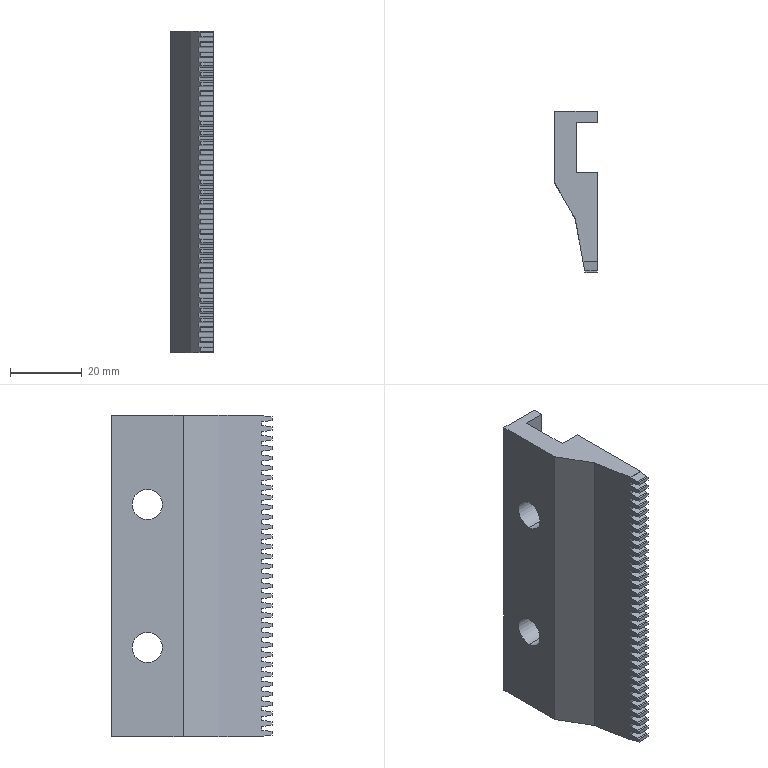Component | SolidWorks | HotKnife.1-1 | 1 solid | 214 faces | box 12 x 45 x 90 mm | volume 27602 mm3 | plane 210 | cylinder 4 | commonest cylinder face diameters 8.5 x4
build123d program:
from build123d import *

# Parameters (mm, degrees)
BOSS_EXTRUDE1_DEPTH            = 45
F_8_5_8_5_DIAMETER_HOLE1_D     = 8.5
F_8_5_8_5_DIAMETER_HOLE1_DEPTH = 80
F_8_5_8_5_DIAMETER_HOLE1_TIP   = 2.554
CUT_EXTRUDE5_DEPTH             = 5
SKETCH5_W                      = 6
SKETCH5_H                      = 14
CUT_EXTRUDE6_DEPTH             = 65


with BuildPart() as part:
    # Sketch1 → Boss-Extrude1 (new, symmetric)
    with BuildSketch(Plane.XY):
        Polygon((0, 0), (0, 45), (12, 45), (12, 25), (6.226, 15), (3.5, 0), align=None)
    extrude(amount=BOSS_EXTRUDE1_DEPTH, both=True)

    # 8.5 _8.5_ Diameter Hole1
    with Locations(Plane(origin=(12, -0.7432, -35.624), x_dir=(0, 0, 1), z_dir=(1, 0, 0))):
        with Locations((15.624, -35.743), (55.624, -35.743)):
            Hole(F_8_5_8_5_DIAMETER_HOLE1_D / 2, depth=F_8_5_8_5_DIAMETER_HOLE1_DEPTH)
            with Locations((0, 0, -(F_8_5_8_5_DIAMETER_HOLE1_DEPTH + F_8_5_8_5_DIAMETER_HOLE1_TIP / 2))):  # 118° drill point
                Cone(0, F_8_5_8_5_DIAMETER_HOLE1_D / 2, F_8_5_8_5_DIAMETER_HOLE1_TIP, mode=Mode.SUBTRACT)

    # Sketch4 → Cut-Extrude5 (cut)
    with BuildSketch(Plane(origin=(0, 0, 0), x_dir=(0, 0, -1), z_dir=(1, 0, 0))):
        Polygon((4.625, 3), (5, 0.5), (5, 0), (6, 0), (6, 0.5), (6.375, 3), (7.375, 3), (7.75, 0.5), (7.75, 0), (8.75, 0), (8.75, 0.5), (9.125, 3), (10.125, 3), (10.5, 0.5), (10.5, 0), (11.5, 0), (11.5, 0.5), (11.875, 3), (12.875, 3), (13.25, 0.5), (13.25, 0), (14.25, 0), (14.25, 0.5), (14.625, 3), (15.625, 3), (16, 0.5), (16, 0), (17, 0), (17, 0.5), (17.375, 3), (18.375, 3), (18.75, 0.5), (18.75, 0), (19.75, 0), (19.75, 0.5), (20.125, 3), (21.125, 3), (21.5, 0.5), (21.5, 0), (22.5, 0), (22.5, 0.5), (22.875, 3), (23.875, 3), (24.25, 0.5), (24.25, 0), (25.25, 0), (25.25, 0.5), (25.625, 3), (26.625, 3), (27, 0.5), (27, 0), (28, 0), (28, 0.5), (28.375, 3), (29.375, 3), (29.75, 0.5), (29.75, 0), (30.75, 0), (30.75, 0.5), (31.125, 3), (32.125, 3), (32.5, 0.5), (32.5, 0), (33.5, 0), (33.5, 0.5), (33.875, 3), (34.875, 3), (35.25, 0.5), (35.25, 0), (36.25, 0), (36.25, 0.5), (36.625, 3), (37.625, 3), (38, 0.5), (38, 0), (39, 0), (39, 0.5), (39.375, 3), (40.375, 3), (40.75, 0.5), (40.75, 0), (41.75, 0), (41.75, 0.5), (42.125, 3), (43.125, 3), (43.5, 0.5), (43.5, 0), (44.5, 0), (44.5, 0.5), (44.875, 3), (45.875, 3), (46.25, 0.5), (46.25, -4.536), (-46.25, -4.536), (-46.25, 0.5), (-45.875, 3), (-44.875, 3), (-44.5, 0.5), (-44.5, 0), (-43.5, 0), (-43.5, 0.5), (-43.125, 3), (-42.125, 3), (-41.75, 0.5), (-41.75, 0), (-40.75, 0), (-40.75, 0.5), (-40.375, 3), (-39.375, 3), (-39, 0.5), (-39, 0), (-38, 0), (-38, 0.5), (-37.625, 3), (-36.625, 3), (-36.25, 0.5), (-36.25, 0), (-35.25, 0), (-35.25, 0.5), (-34.875, 3), (-33.875, 3), (-33.5, 0.5), (-33.5, 0), (-32.5, 0), (-32.5, 0.5), (-32.125, 3), (-31.125, 3), (-30.75, 0.5), (-30.75, 0), (-29.75, 0), (-29.75, 0.5), (-29.375, 3), (-28.375, 3), (-28, 0.5), (-28, 0), (-27, 0), (-27, 0.5), (-26.625, 3), (-25.625, 3), (-25.25, 0.5), (-25.25, 0), (-24.25, 0), (-24.25, 0.5), (-23.875, 3), (-22.875, 3), (-22.5, 0.5), (-22.5, 0), (-21.5, 0), (-21.5, 0.5), (-21.125, 3), (-20.125, 3), (-19.75, 0.5), (-19.75, 0), (-18.75, 0), (-18.75, 0.5), (-18.375, 3), (-17.375, 3), (-17, 0.5), (-17, 0), (-16, 0), (-16, 0.5), (-15.625, 3), (-14.625, 3), (-14.25, 0.5), (-14.25, 0), (-13.25, 0), (-13.25, 0.5), (-12.875, 3), (-11.875, 3), (-11.5, 0.5), (-11.5, 0), (-10.5, 0), (-10.5, 0.5), (-10.125, 3), (-9.125, 3), (-8.75, 0.5), (-8.75, 0), (-7.75, 0), (-7.75, 0.5), (-7.375, 3), (-6.375, 3), (-6, 0.5), (-6, 0), (-5, 0), (-5, 0.5), (-4.625, 3), (-3.625, 3), (-3.25, 0.5), (-3.25, 0), (-2.25, 0), (-2.25, 0.5), (-1.875, 3), (-0.875, 3), (-0.5, 0.5), (-0.5, 0), (0.5, 0), (0.5, 0.5), (0.875, 3), (1.875, 3), (2.25, 0.5), (2.25, 0), (3.25, 0), (3.25, 0.5), (3.625, 3), align=None)
    extrude(amount=CUT_EXTRUDE5_DEPTH, mode=Mode.SUBTRACT)

    # Sketch5 → Cut-Extrude6 (cut, symmetric)
    with BuildSketch(Plane.XY):
        with Locations((3, 35)):
            Rectangle(SKETCH5_W, SKETCH5_H)
    extrude(amount=CUT_EXTRUDE6_DEPTH, both=True, mode=Mode.SUBTRACT)


solid = part.part

# Placed as in the assembly
solid = solid.moved(Location((-5.75, 156, 0), (-180, 0, 180)))